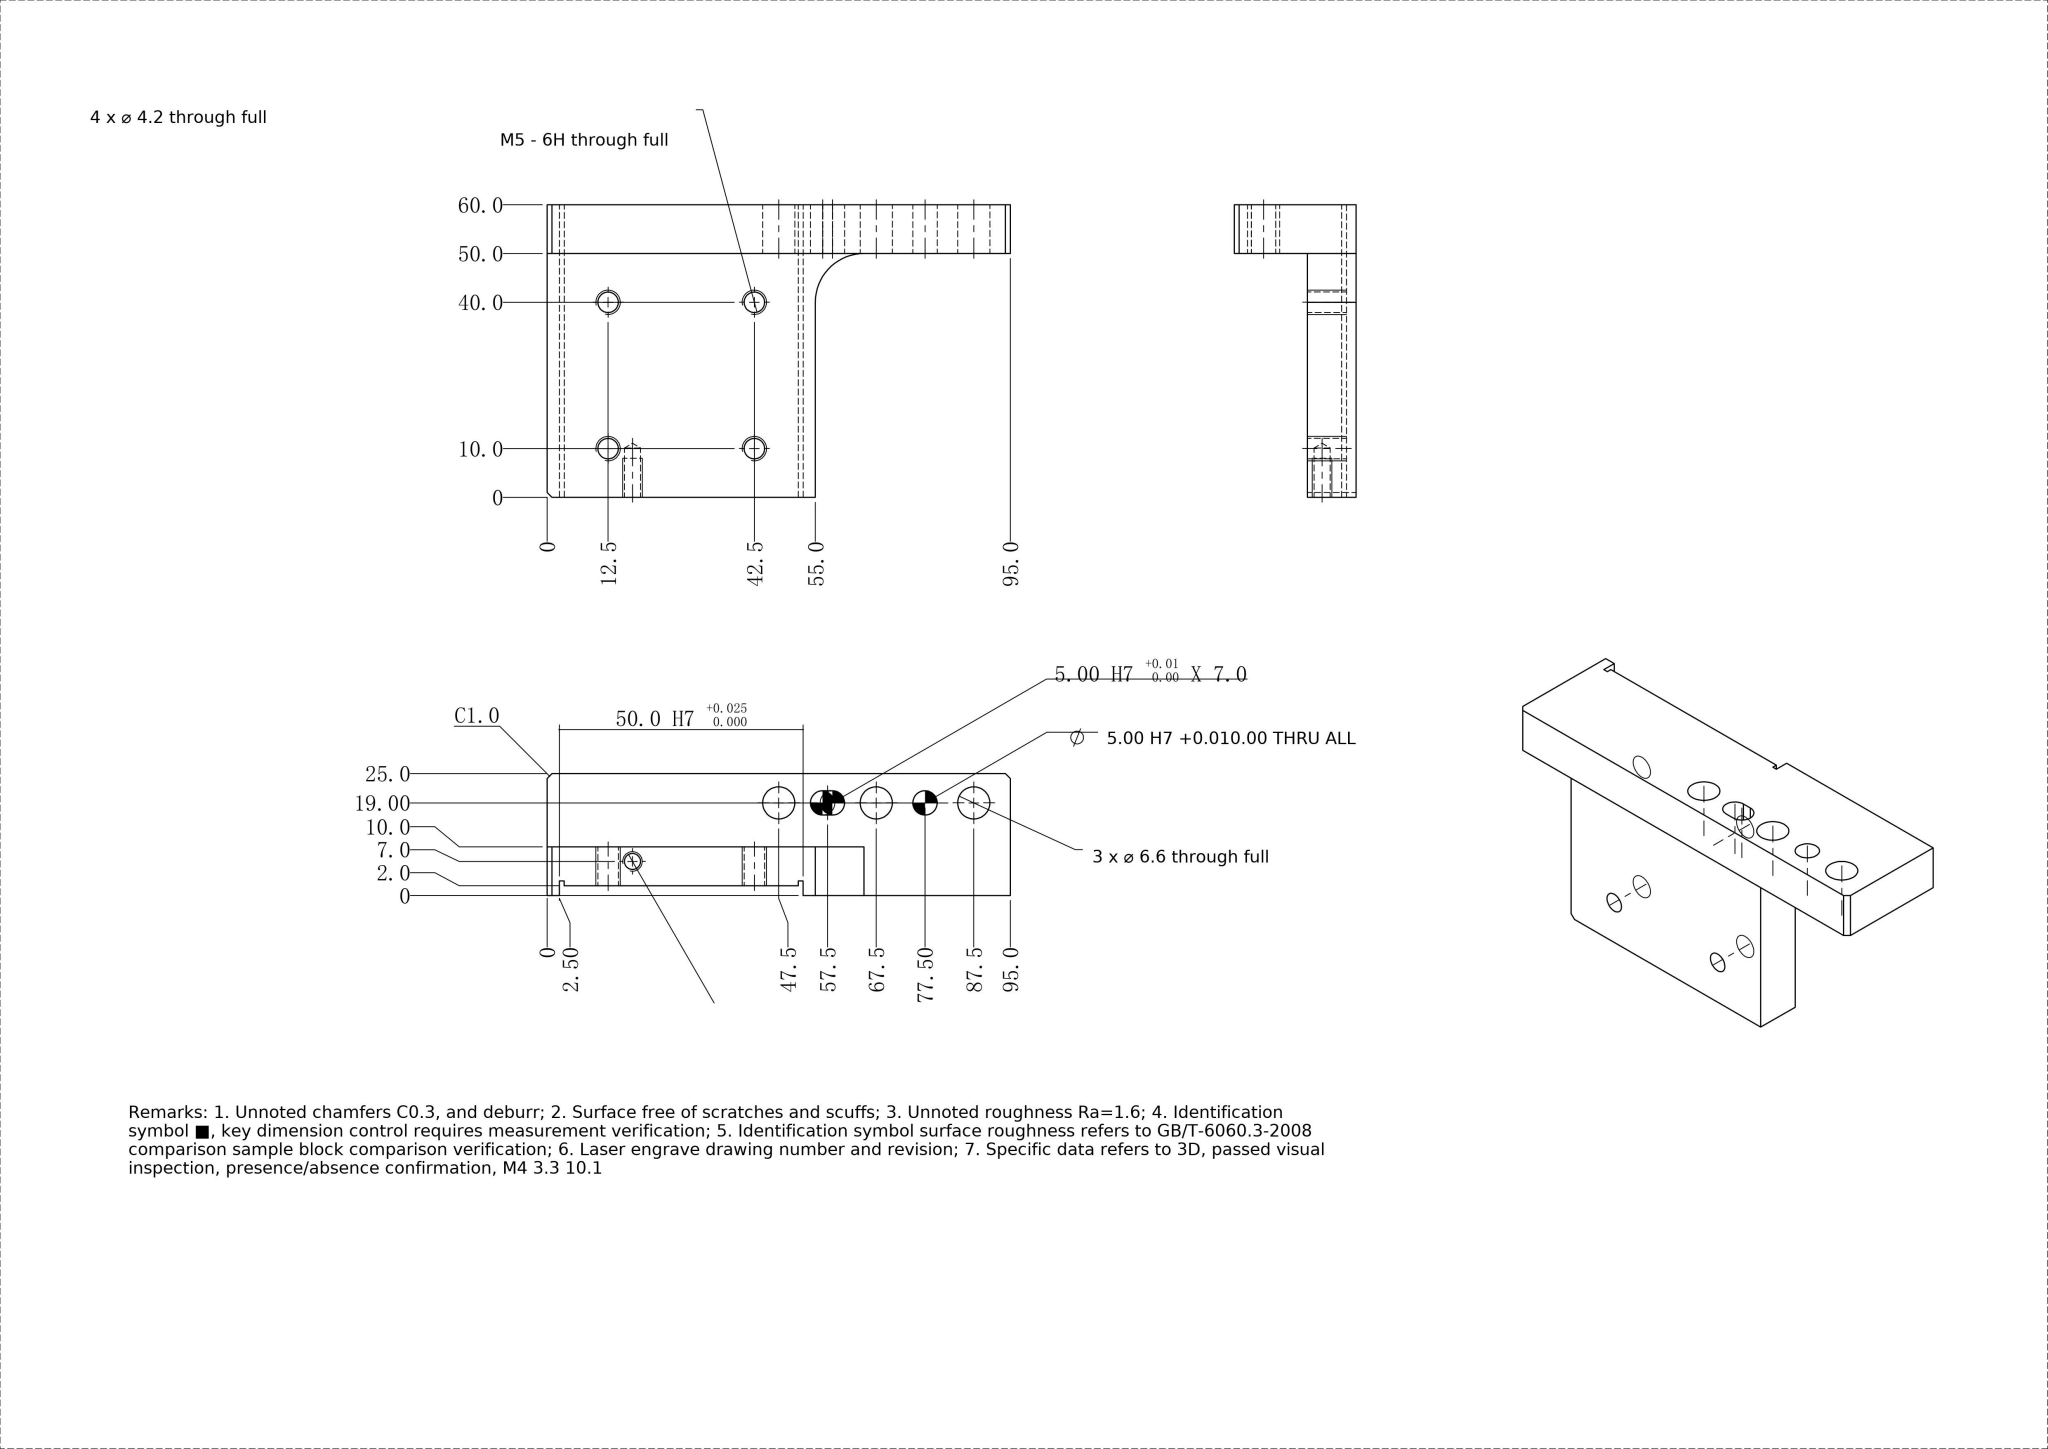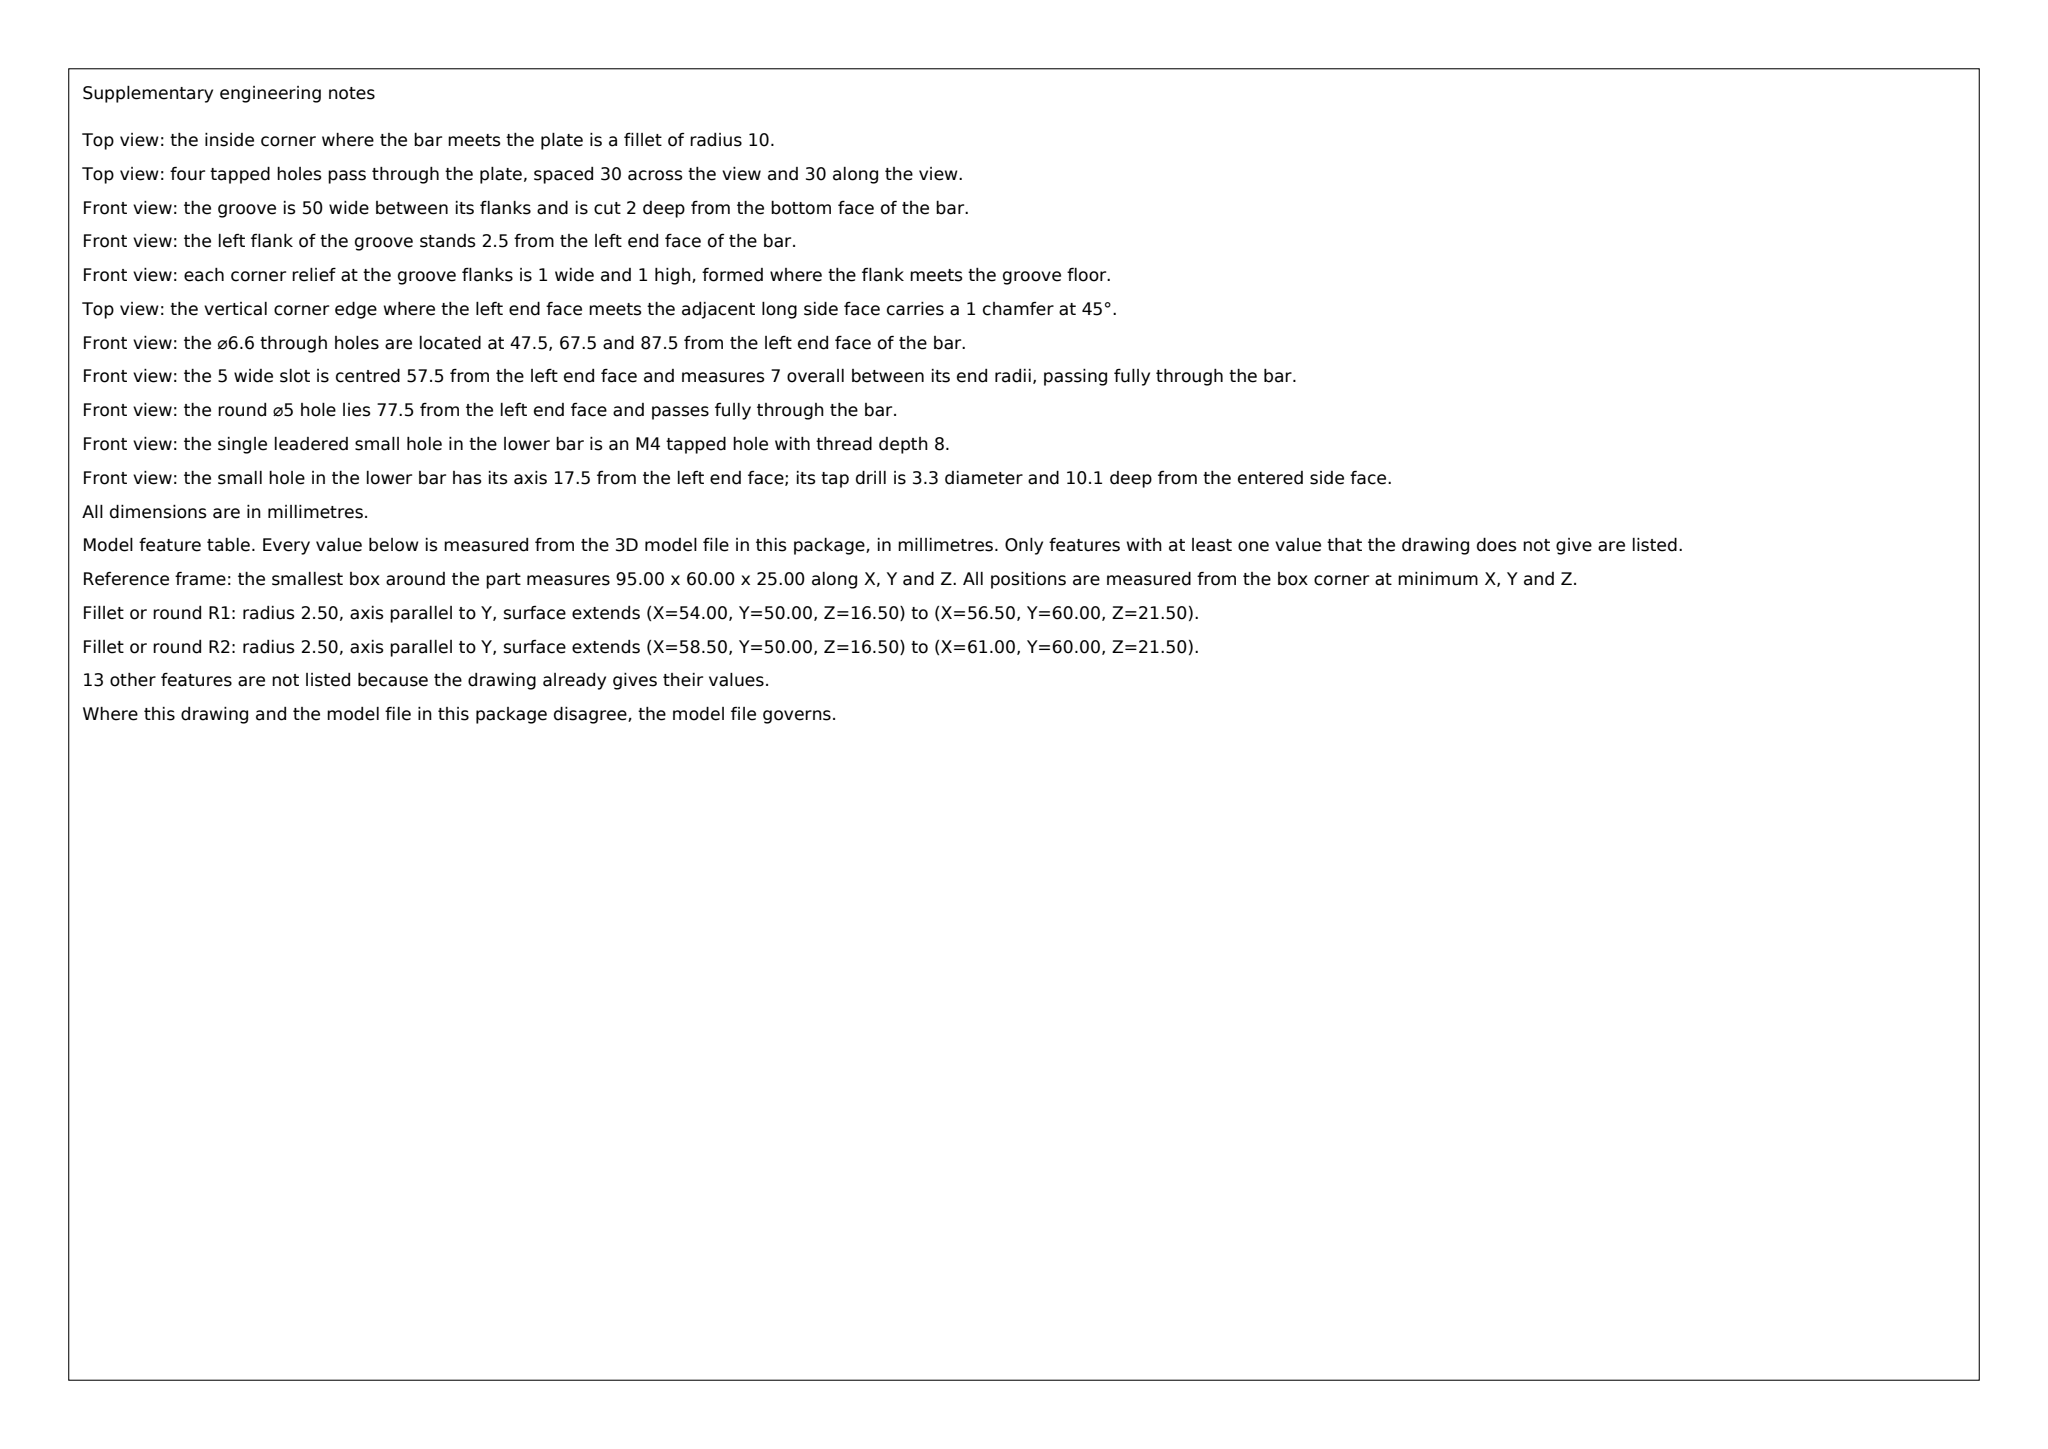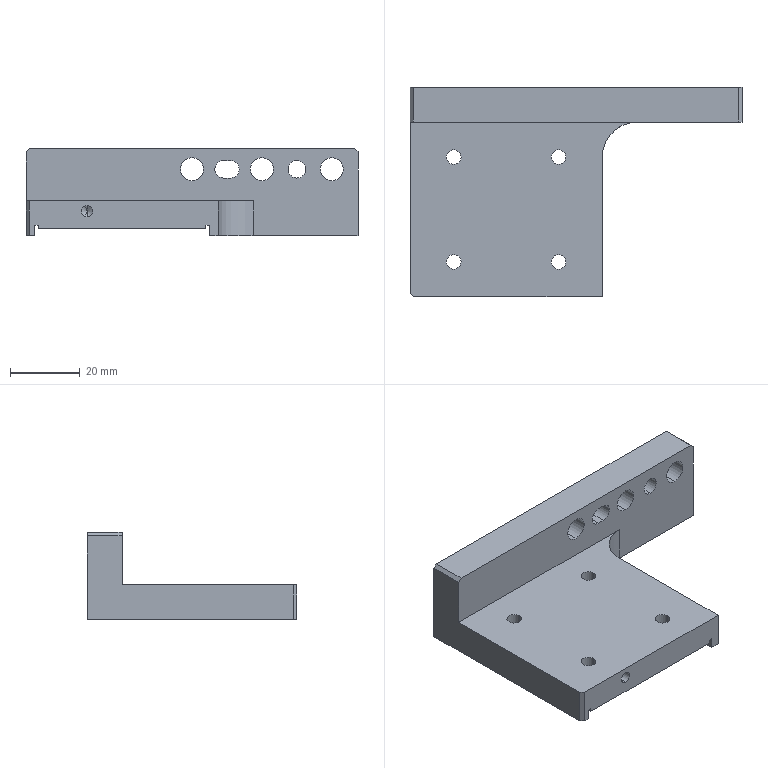Part | SolidWorks | mm | 1 solid | 46 faces | box 95 x 60 x 25 mm | volume 43278 mm3 | cylinder 22 | plane 22 | cone 2 | commonest cylinder face diameters 4.2 x8 6.6 x6 5 x5 3.3 x2 20 x1
Drawing notes:
VERT RIB THK 8.0, Z2.0 TO Z10.0, X0 TO X55, Y0 TO Y50 | from the solid: z planes 2.0/10.0 (8 apart), x 0/55, y 0/50; 4X O4.2 z-holes length 8.0
TAPPED HOLE: M4 (Ø3.3 TAP DRILL) AT X17.5, Z7.0; DRILLED FROM Y0 FACE, 10.1 DEEP (BLIND, NOT THRU), 118° DRILL POINT | from the solid: cylinders: hole/bore dia 3.3, axis y at [17.5, -, 7.0], from y=0.0 to 10.1; cones 118° ref_dia 3.3 at y=10.1
2X 1.0 WIDE X 1.0 DEEP RELIEF GROOVE IN RIB BOTTOM, FULL WIDTH Y0 TO Y60: GROOVE 1 WALLS AT X2.5 AND X3.5; GROOVE 2 WALLS AT X51.5 AND X52.5 (FROM X0 DATUM); GROOVE FLOORS AT Z3.0, RIB UNDERSIDE AT Z2.0 | from the solid: axis_planes x=2.5, x=3.5, x=51.5, x=52.5 (z 0-3 / 2-3) and z=3.0 planes x[2.5-3.5] and x[51.5-52.5]; z=2.0 plane x[3.5-51.5]